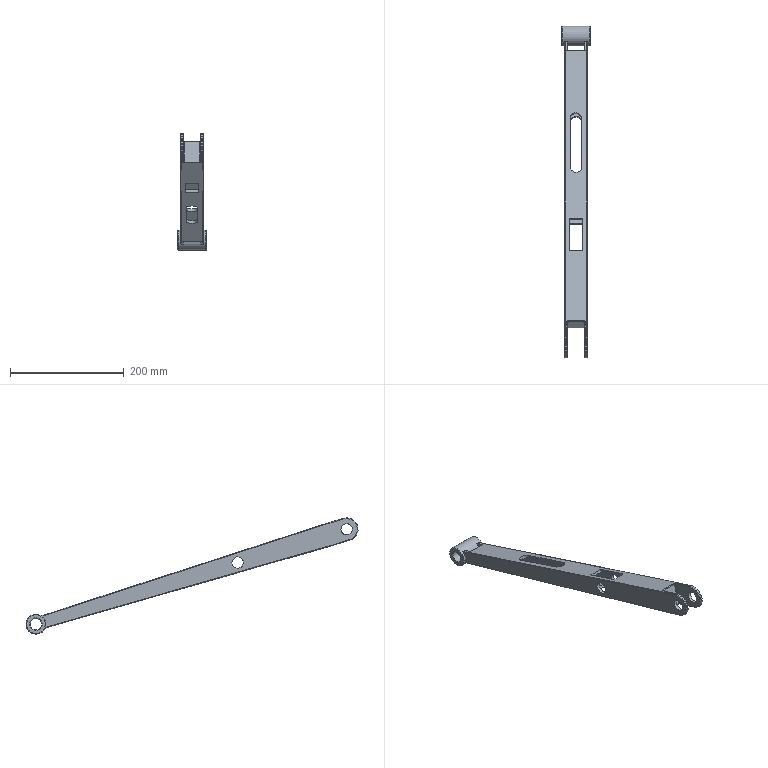Component | NX | CCJ-005 | 1 solid | 96 faces | volume 326198 mm3 | plane 36 | cylinder 36 | torus 12 | sphere 8 | spline 4 | commonest cylinder face diameters 2 x24 20 x9 40 x2 35 x1